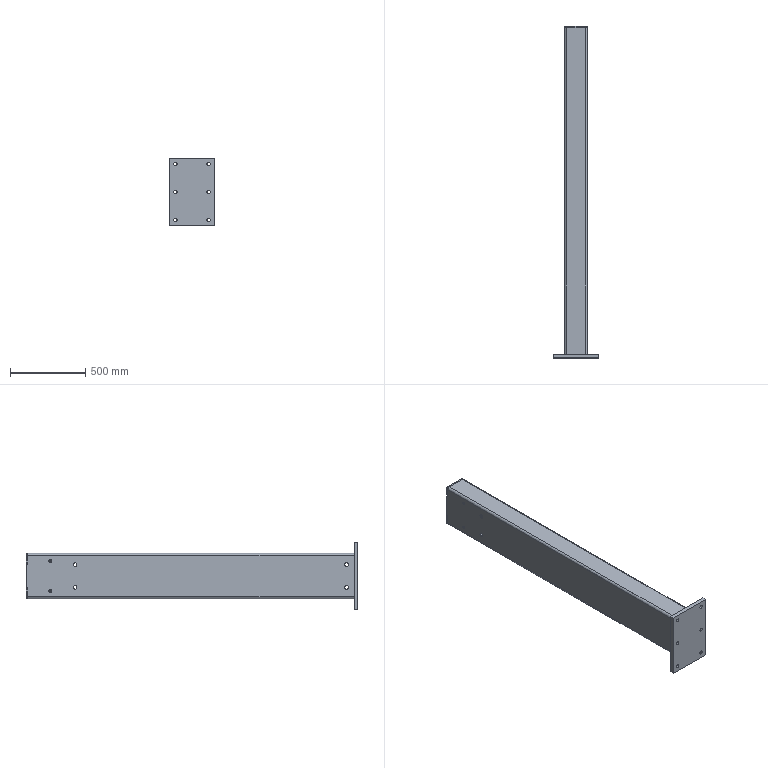Component | NX | COLUMN | 3 solids | 70 faces | volume 12748400 mm3 | plane 37 | cylinder 29 | cone 4 | commonest cylinder face diameters 28 x10 22 x6 16 x6 25 x4 17.5 x2 50 x1